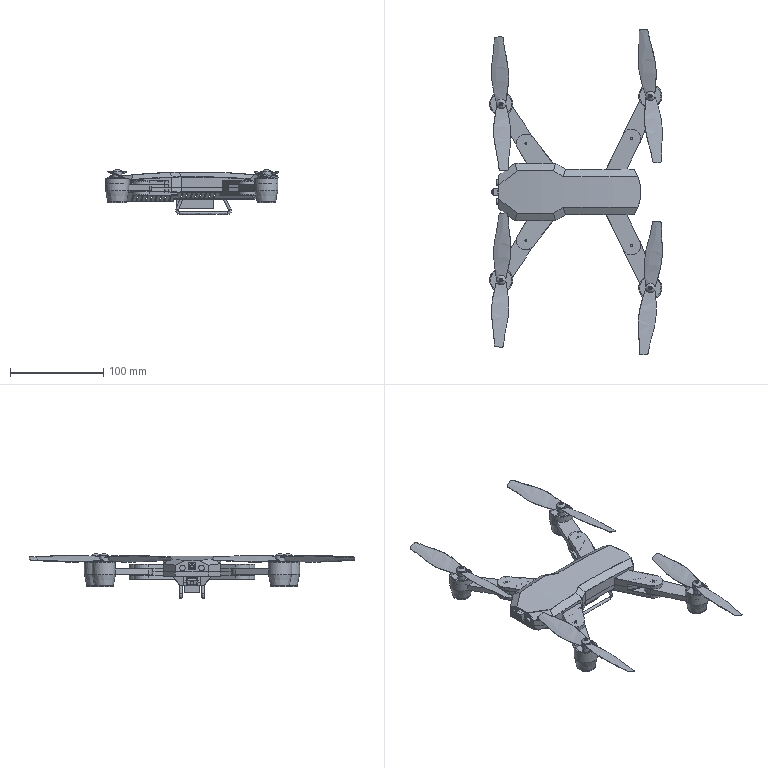Assembly | NX | mm | 29 component files | 29 solids | 1003 faces | box 185.79 x 350.1 x 48.23 mm | volume 114346 mm3 | plane 602 | cylinder 278 | spline 81 | cone 22 | torus 20 | commonest cylinder face diameters 2 x81 1.5 x68 4 x17 20 x16 6 x11 3.8 x8 2.2 x8 18 x8
Bill of materials:
unnamed part 1 | 4 |  | Two-blade, propeller-like rotor: a central cylindrical hub with a domed top and a small axial hole, and two long, thin, twisted blades on opposite sides.
unnamed part 2 | 1 |  | Rounded rectangular block body with a cylindrical shaft sticking out from the center of each opposite end face.
unnamed part 3 | 4 |  | Socket-head-cap-screw-like fastener: a cylindrical head with a hexagonal recess and a plain cylindrical shank.
unnamed part 4 | 2 |  | Short stepped cylindrical pin: a wide, short cylindrical head with a narrower, longer coaxial shaft.
unnamed part 5 | 4 |  | Thin flat circular disc of uniform thickness.
unnamed part 6 | 1 |  | Thin flat plate: a rectangular main region joined to a wider end tab whose outer edge is a convex arc.
unnamed part 7 | 1 |  | X-shaped frame-like base: an elongated central tray with four angled arms ending in rounded pads, each pad with a small hole and a raised boss.
unnamed part 8 | 2 |  | Large solid cylinder with a smaller coaxial cylindrical boss sticking out from one flat end face.
unnamed part 9 | 4 |  | Long, slender headed pin: a short cylindrical head with a long, thin coaxial shank.
unnamed part 10 | 1 |  | Shell or cover with the same X-shaped outline as a four-arm frame: a raised elongated central body with chamfered and faceted edges, and four flat arms ending in rounded pads with small holes.
unnamed part 11 | 4 |  | Lever-like part: a flat bar with rounded ends, one end carrying a hole and the other end joined to an open cylindrical cup that has a hexagonal central post with an axial hole.
unnamed part 12 | 1 |  | Rectangular block with a rectangular slot cut through one side, plus a two-step cylindrical boss on one face.
Mates:
1. fix | lower_housing 1 component
2. touch align | upper_housing 1 face | lower_housing 1 face
3. touch align | upper_housing 1 face | lower_housing 1 face
4. touch align | upper_housing 1 face | lower_housing 1 face
5. concentric | propeller_bracket 2 edge | upper_housing 1 edge
6. parallel | propeller_bracket 2 face | upper_housing 1 face
7. concentric | propeller_bracket 1 edge | upper_housing 1 edge
8. parallel | propeller_bracket 1 face | upper_housing 1 face
9. concentric | propeller_bracket 4 edge | upper_housing 1 edge
10. parallel | propeller_bracket 4 face | upper_housing 1 face
11. concentric | propeller_bracket 3 edge | upper_housing 1 edge
12. parallel | propeller_bracket 3 face | lower_housing 1 face
13. concentric | M6_screw 4 edge | lower_housing 1
14. concentric | M6_screw 3 edge | lower_housing 1
15. concentric | M6_screw 2 edge | lower_housing 1
16. concentric | M3_screw 1 edge | lower_housing 1 edge
17. concentric | M3_screw 2 edge | lower_housing 1 edge
18. concentric | M6_screw 1 edge | lower_housing 1 edge
19. concentric | propeller 3 edge | propeller_bracket 1 edge
20. concentric | propeller 4 edge | propeller_bracket 2 edge
21. concentric | propeller 1 edge | propeller_bracket 3 edge
22. concentric | propeller 2 edge | propeller_bracket 4 edge
23. concentric | M2X10_screw 4 edge | propeller 1 edge
24. concentric | M2X10_screw 3 edge | propeller 2 edge
25. concentric | M2X10_screw 1 edge | propeller 4 edge
26. concentric | M2X10_screw 2 edge | propeller 3 edge
27. touch align | battery_cover 1 face | lower_housing 1 face
28. touch align | battery_cover 1 face | lower_housing 1 face
29. touch align | battery_cover 1 face | lower_housing 1 face
30. concentric | camera 1 edge | lower_housing 1 edge
31. touch align | IR_thermal_imager 1 face | upper_housing 1 face
32. concentric | LED_light 2 edge | upper_housing 1 edge
33. concentric | LED_light 1 edge | upper_housing 1 edge
34. concentric | damping_pad_2 4 edge | propeller_bracket 1 edge
35. concentric | damping_pad_2 1 edge | propeller_bracket 2 edge
36. concentric | damping_pad_2 2 edge | propeller_bracket 3 edge
37. concentric | damping_pad_2 3 edge | propeller_bracket 4 edge